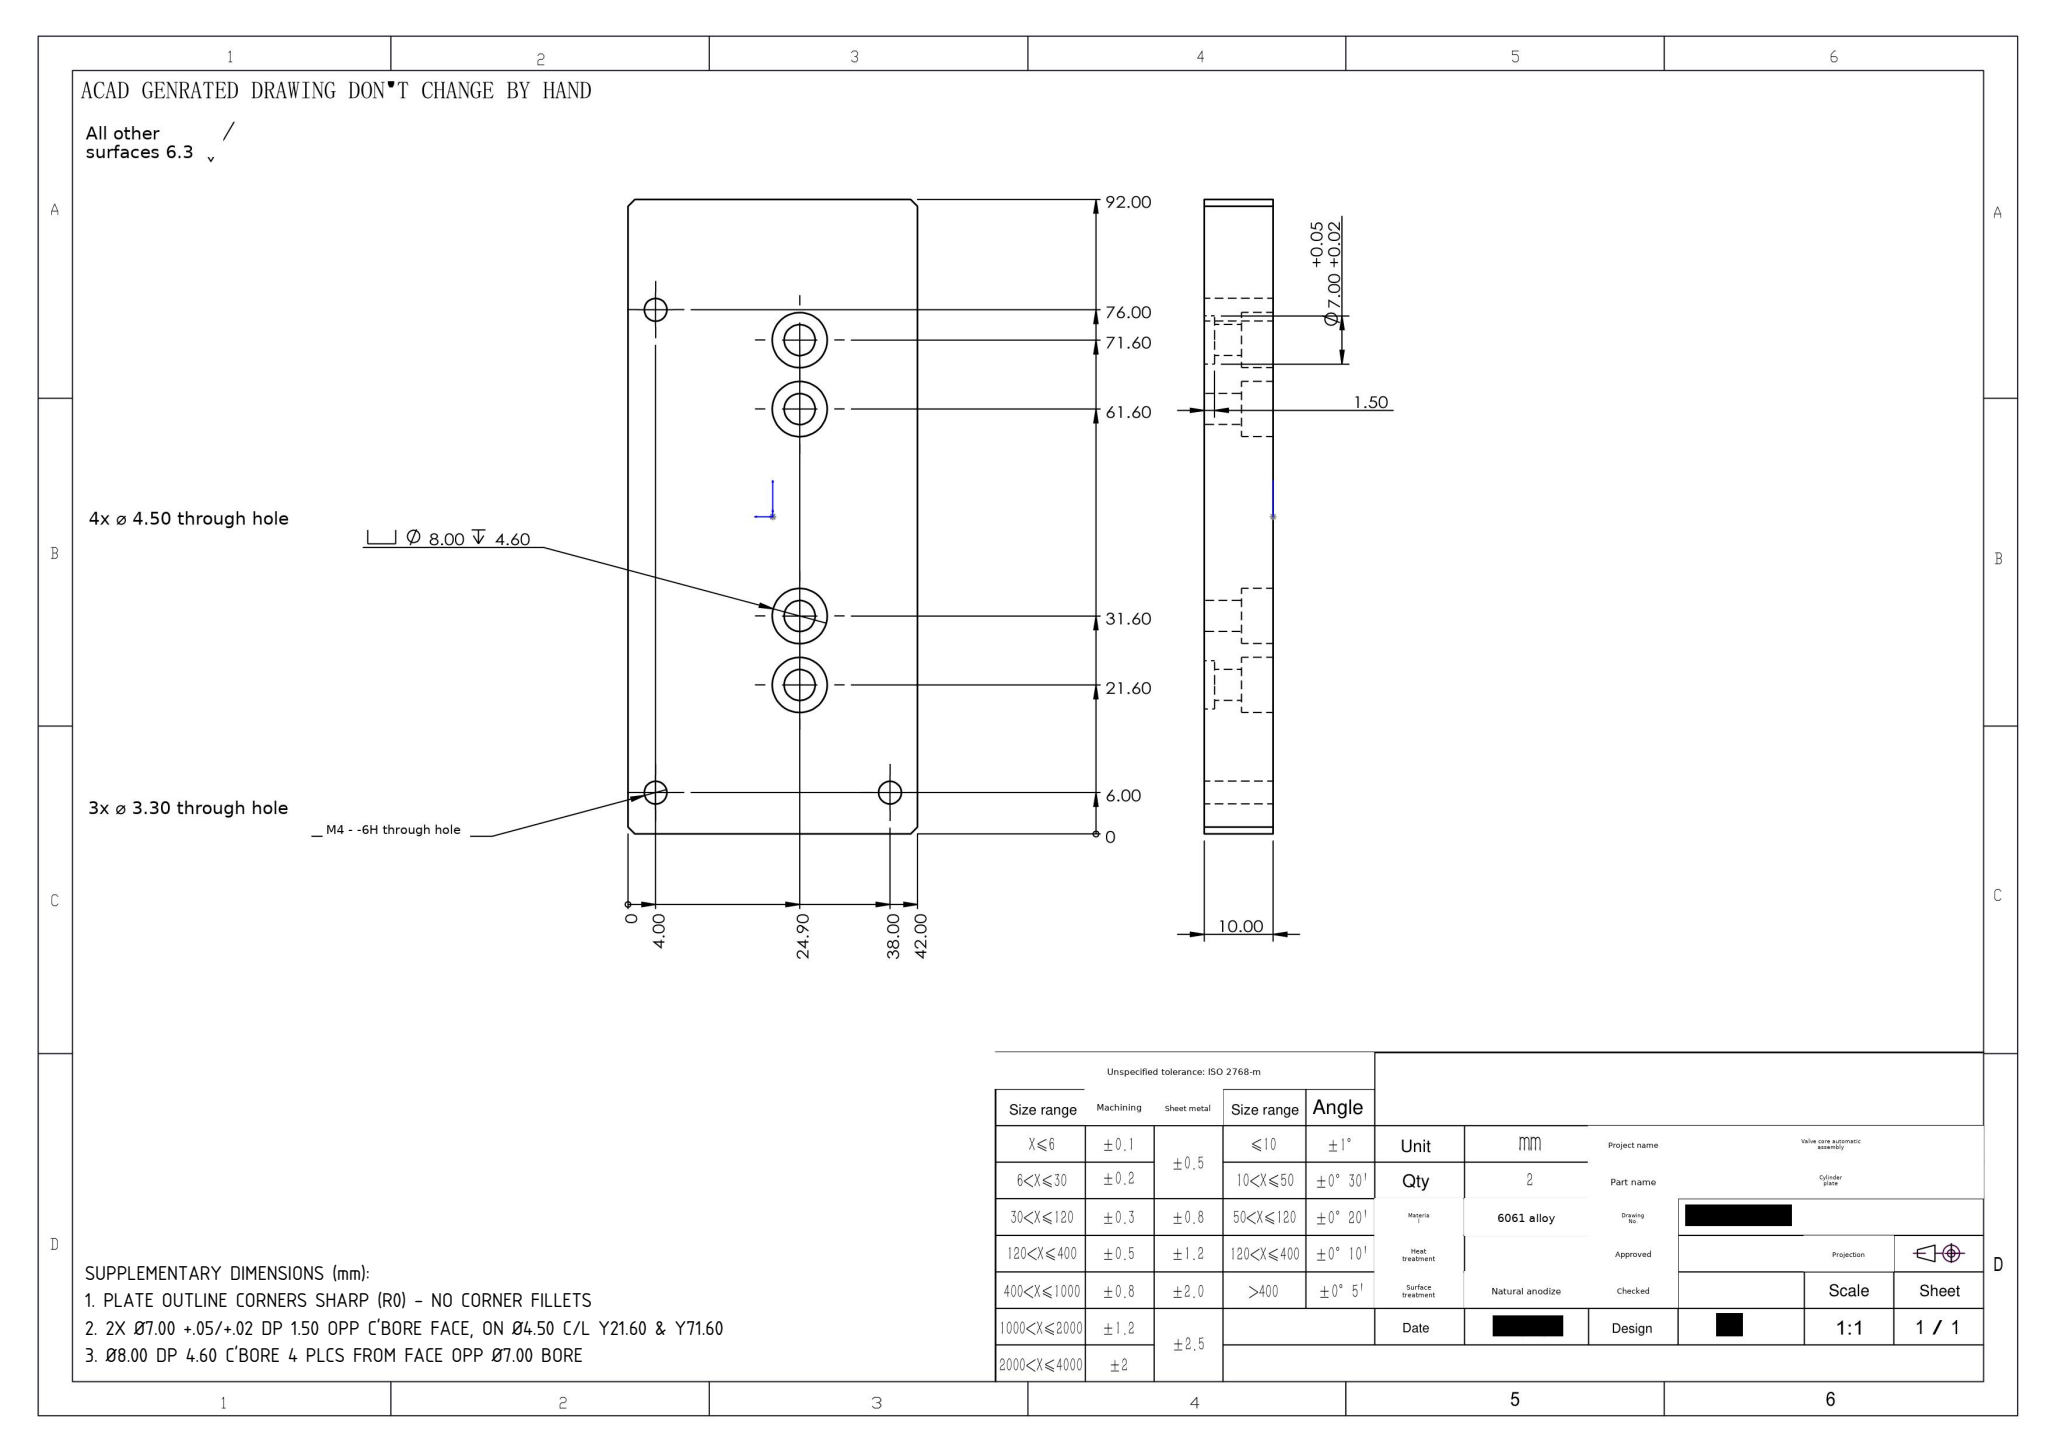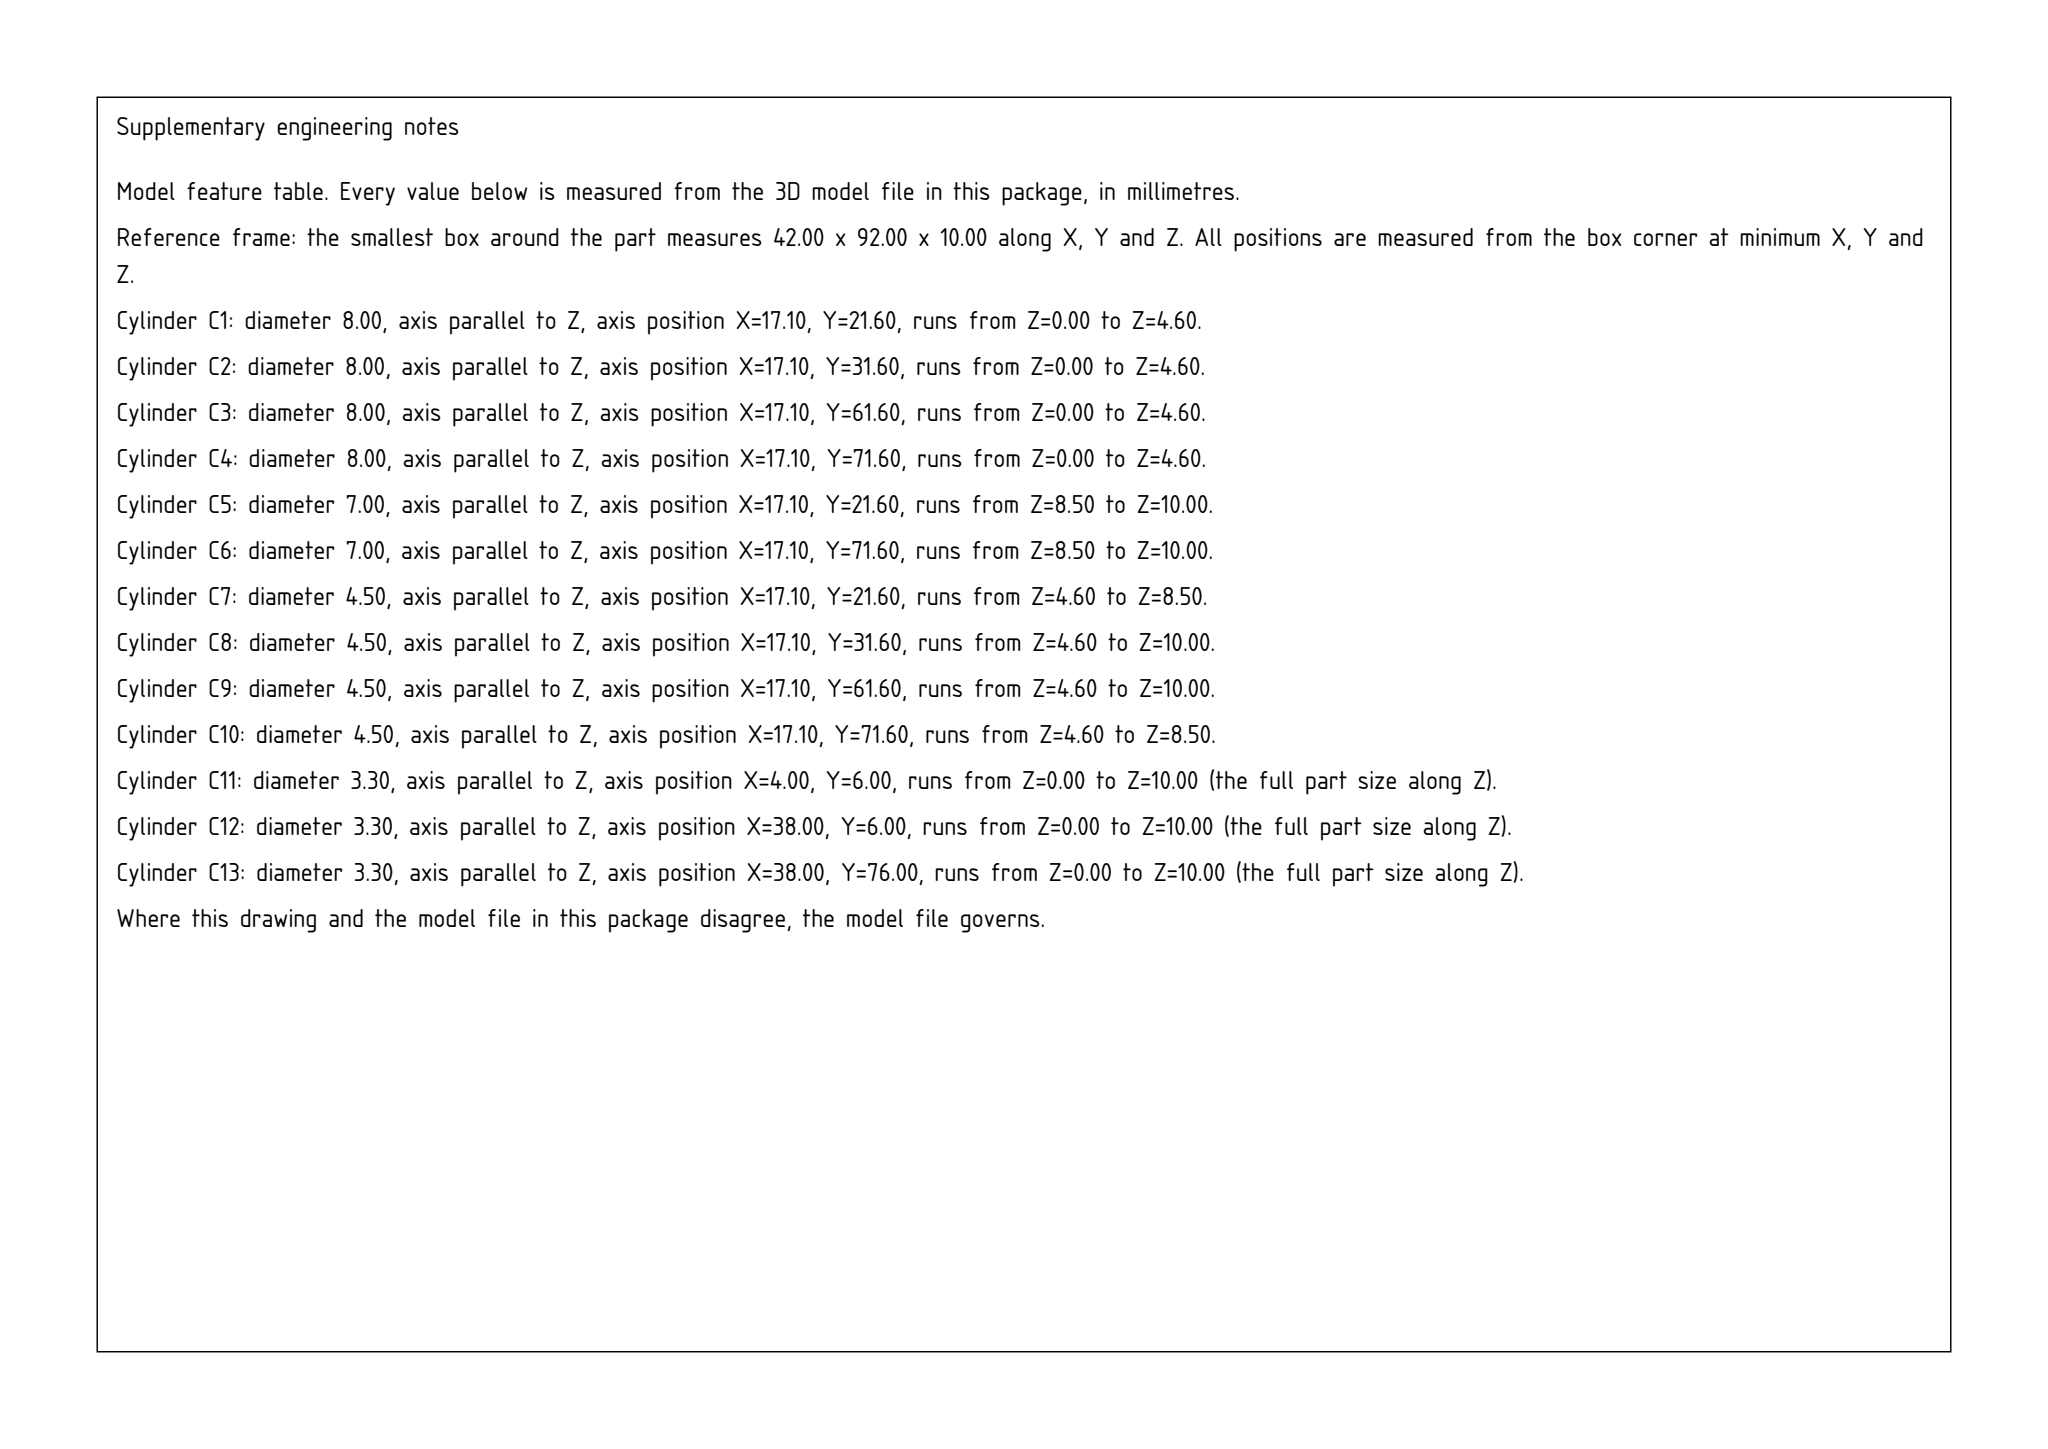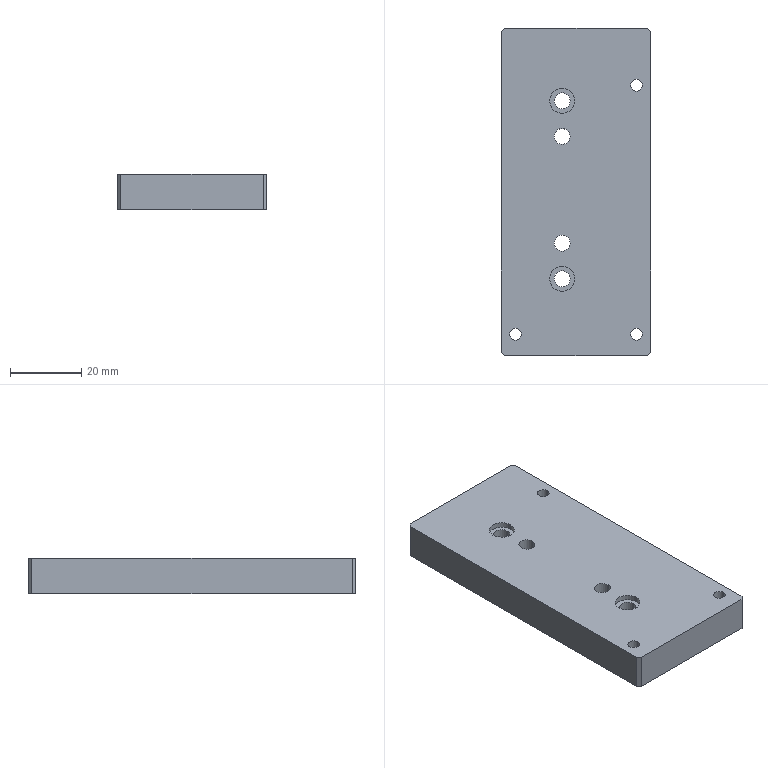Part | SolidWorks | mm | 1 solid | 42 faces | box 42 x 92 x 10 mm | volume 37027 mm3 | cylinder 26 | plane 16 | commonest cylinder face diameters 8 x8 4.5 x8 3.3 x6 7 x4
build123d program:
from build123d import *

# Parameters (mm, degrees)
SKETCH2_W                                           = 42
SKETCH2_H                                           = 92
BOSS_EXTRUDE1_DEPTH                                 = 10
CYLINDRICAL_COUNTERSUNK_HOLE_FOR_M4_HEX_D           = 4.5
CYLINDRICAL_COUNTERSUNK_HOLE_FOR_M4_HEX_CBORE_D     = 8
CYLINDRICAL_COUNTERSUNK_HOLE_FOR_M4_HEX_CBORE_DEPTH = 4.6
M4_TAPPED_HOLE1_D                                   = 3.3
CHAMFER1_SIZE                                       = 1
SKETCH7_R                                           = 3.5
CUT_EXTRUDE1_DEPTH                                  = 1.5


with BuildPart() as part:
    # Sketch2 → Boss-Extrude1 (new body)
    with BuildSketch(Plane(origin=(0, 0, 0), x_dir=(-1, 0, 0), z_dir=(0, 0, -1))):
        Rectangle(SKETCH2_W, SKETCH2_H)
    extrude(amount=-BOSS_EXTRUDE1_DEPTH)

    # Cylindrical Countersunk Hole for M4 Hex (through all)
    with Locations(Plane(origin=(0, 0, 0), x_dir=(-1, 0, 0), z_dir=(0, 0, -1))):
        with Locations((3.9, -24.4), (3.9, -14.4), (3.9, 15.6), (3.9, 25.6)):
            CounterBoreHole(CYLINDRICAL_COUNTERSUNK_HOLE_FOR_M4_HEX_D / 2, CYLINDRICAL_COUNTERSUNK_HOLE_FOR_M4_HEX_CBORE_D / 2, CYLINDRICAL_COUNTERSUNK_HOLE_FOR_M4_HEX_CBORE_DEPTH)

    # M4 Tapped Hole1 (through all)
    with Locations(Plane(origin=(0, 0, 0), x_dir=(-1, 0, 0), z_dir=(0, 0, -1))):
        with Locations((17, -40), (-17, -40), (-17, 30)):
            Hole(M4_TAPPED_HOLE1_D / 2)

    # Chamfer1
    chamfer1_edges = [part.edges().sort_by_distance(p)[0] for p in [
        (-21, 46, 5),
        (-21, -46, 5),
        (21, -46, 5),
        (21, 46, 5),
    ]]
    chamfer(chamfer1_edges, length=CHAMFER1_SIZE)

    # Sketch7 → Cut-Extrude1 (cut)
    with BuildSketch(Plane.XY.offset(10)):
        with Locations((-3.9, 25.6)):
            Circle(SKETCH7_R)
        with Locations((-3.9, -24.4)):
            Circle(SKETCH7_R)
    extrude(amount=-CUT_EXTRUDE1_DEPTH, mode=Mode.SUBTRACT)


solid = part.part